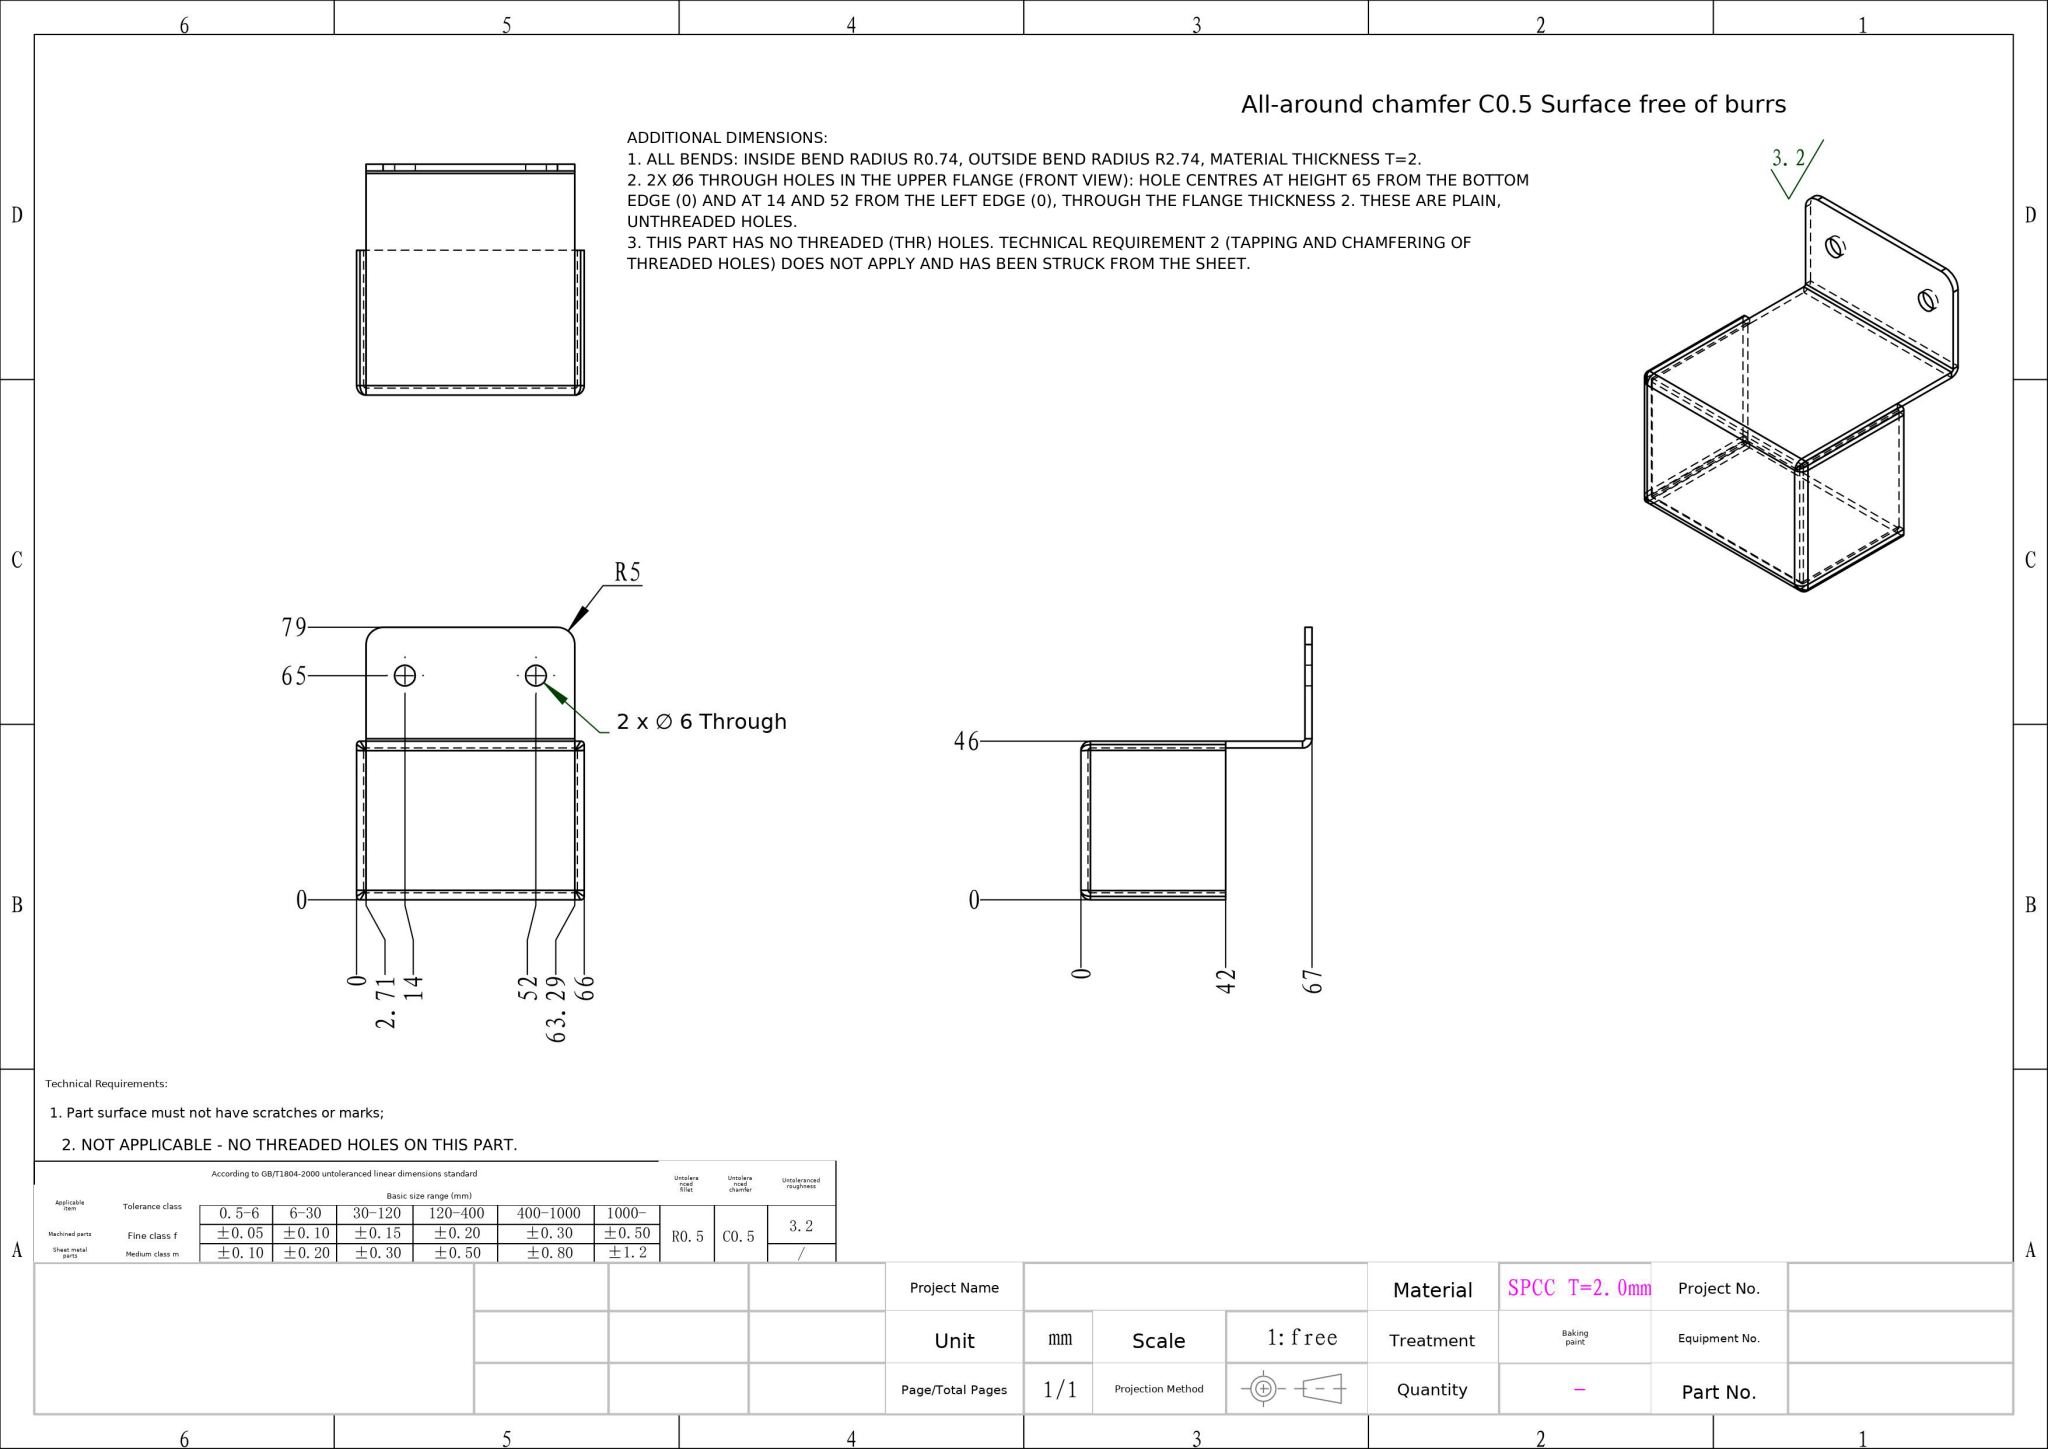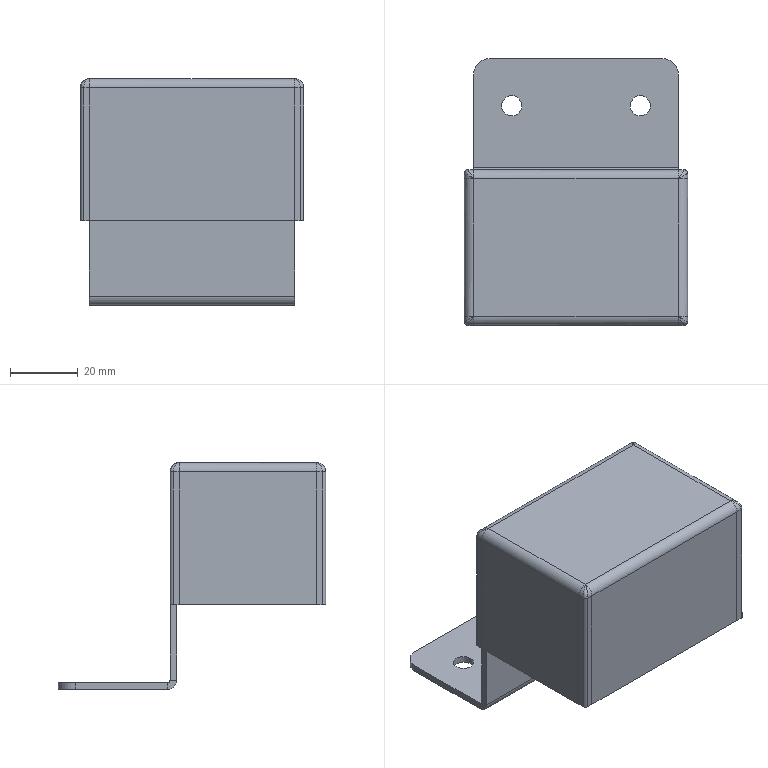Part | NX | mm | 1 solid | 82 faces | box 66 x 79 x 67 mm | volume 29792 mm3 | plane 42 | cylinder 20 | spline 20 | commonest cylinder face diameters 5.473 x5 1.473 x5 6 x4 2 x4 10 x2